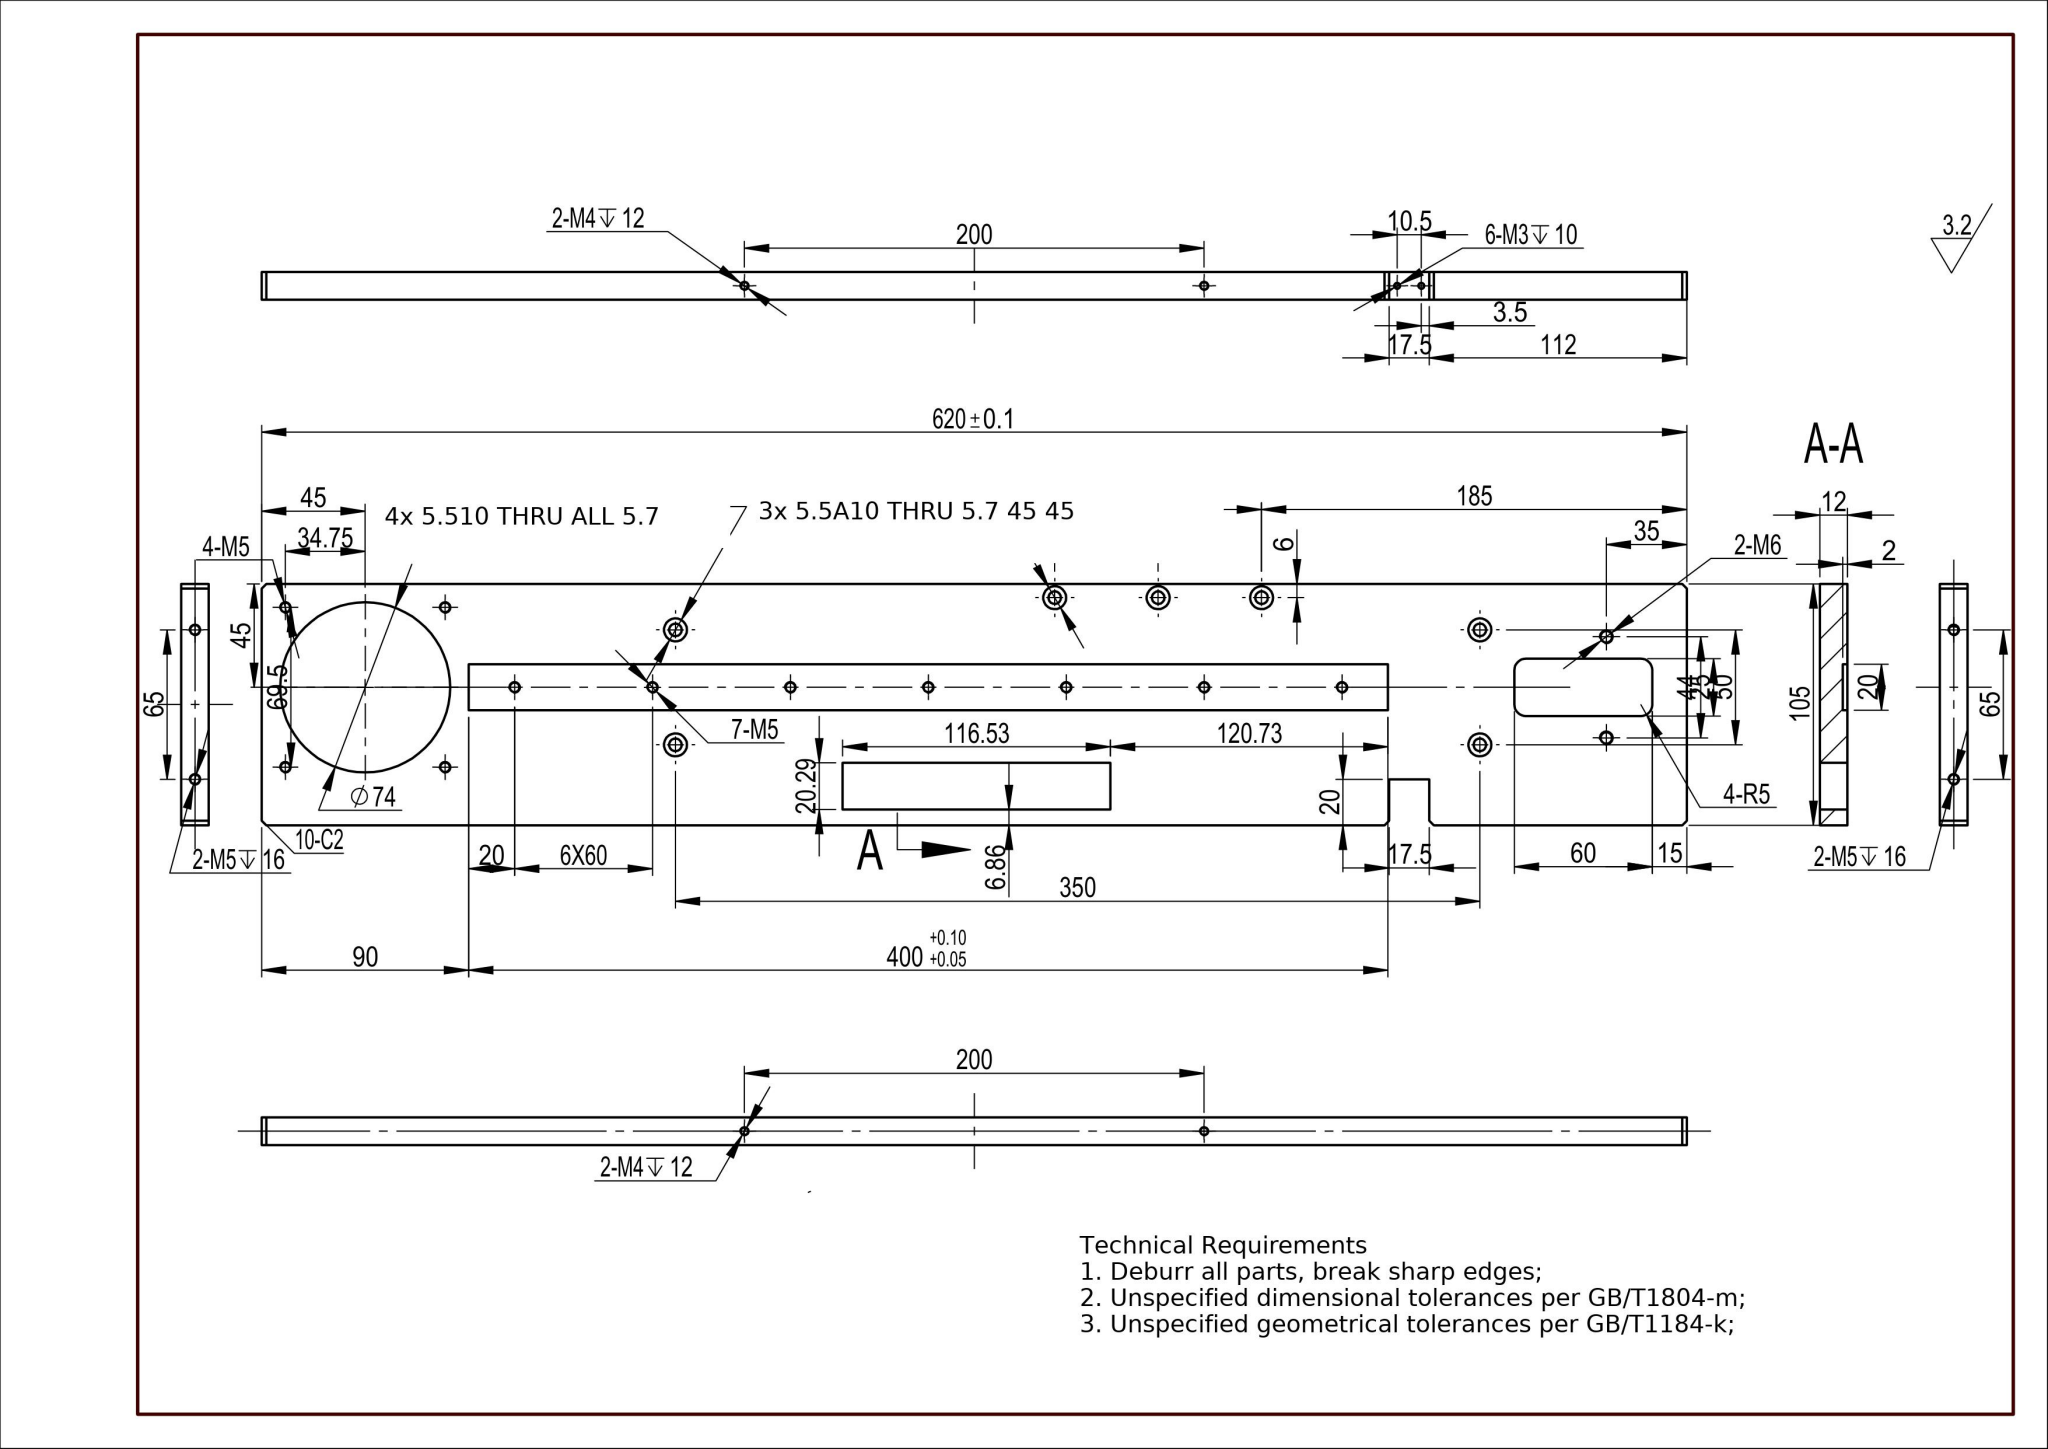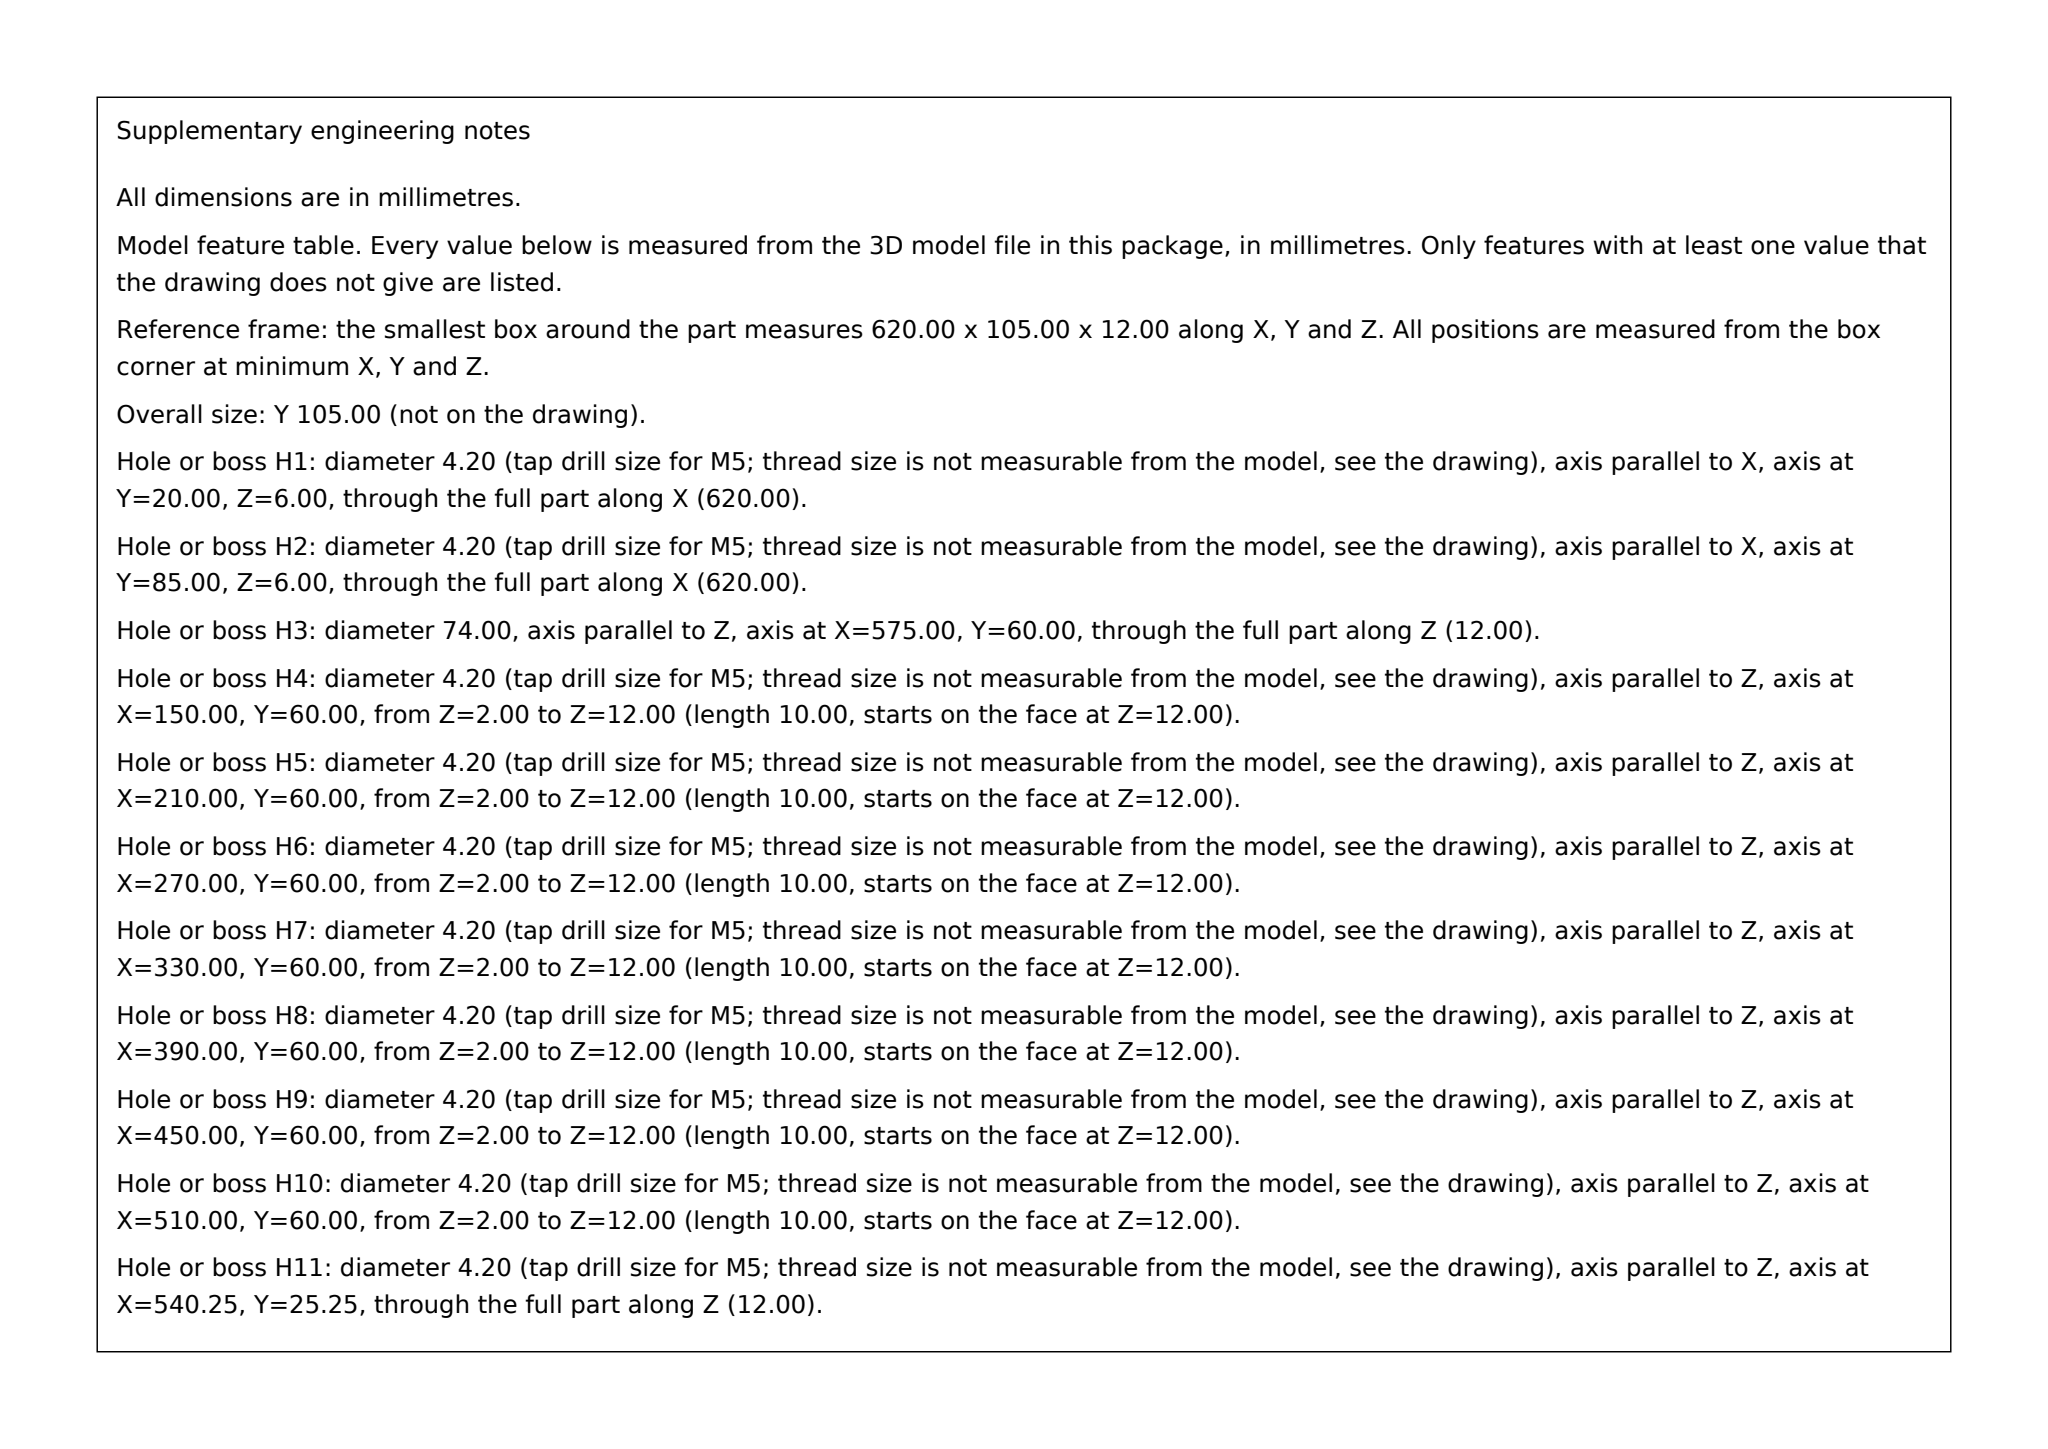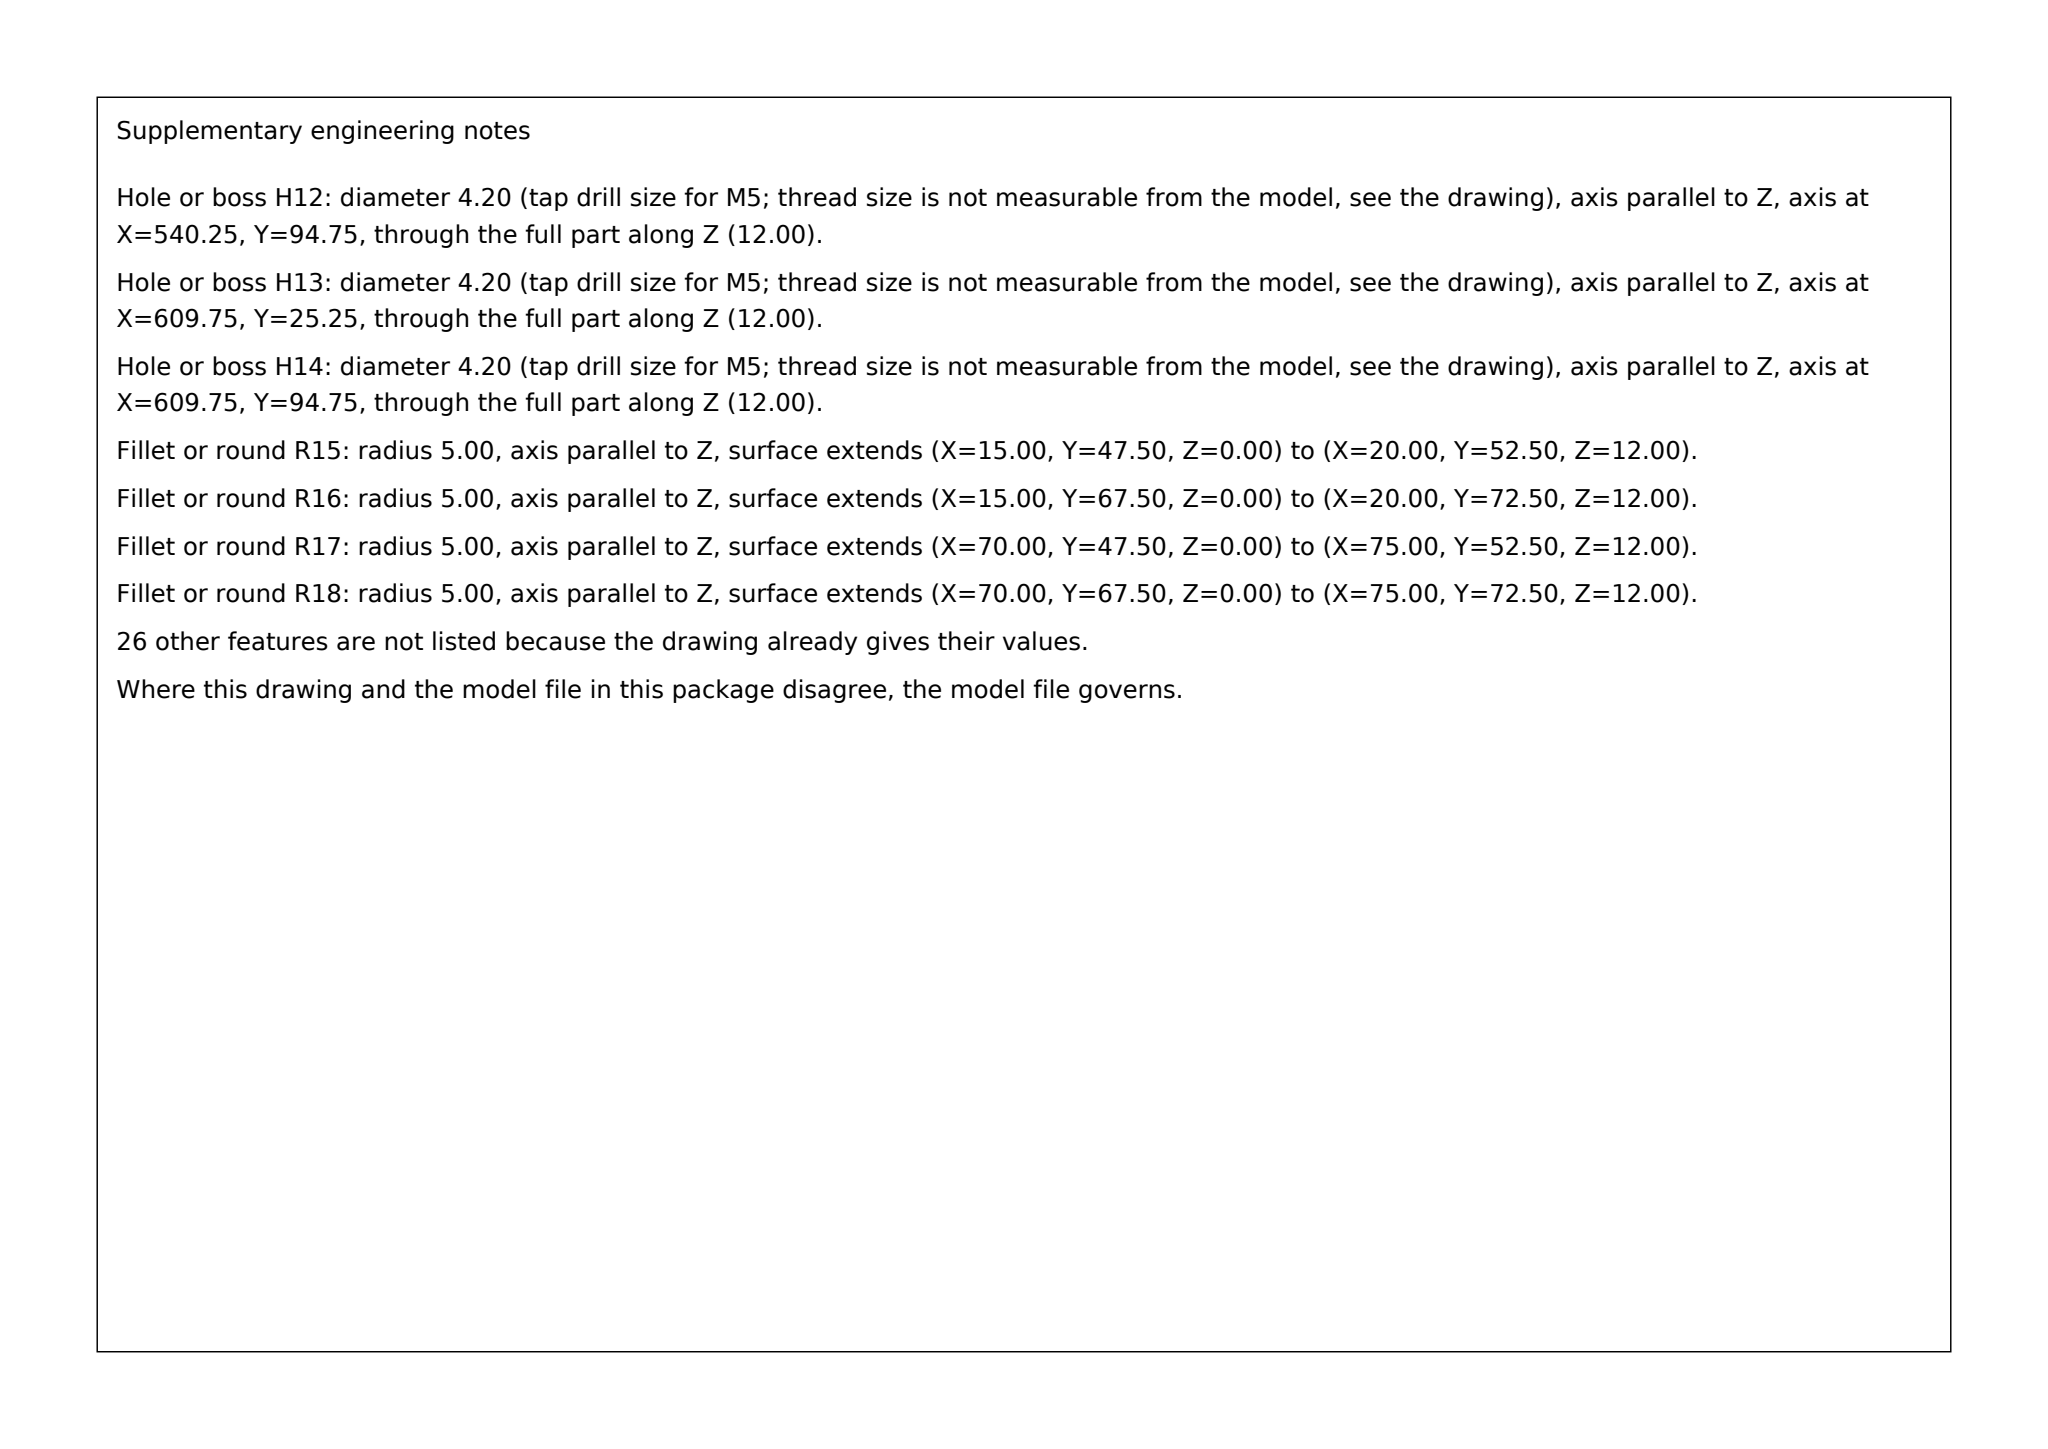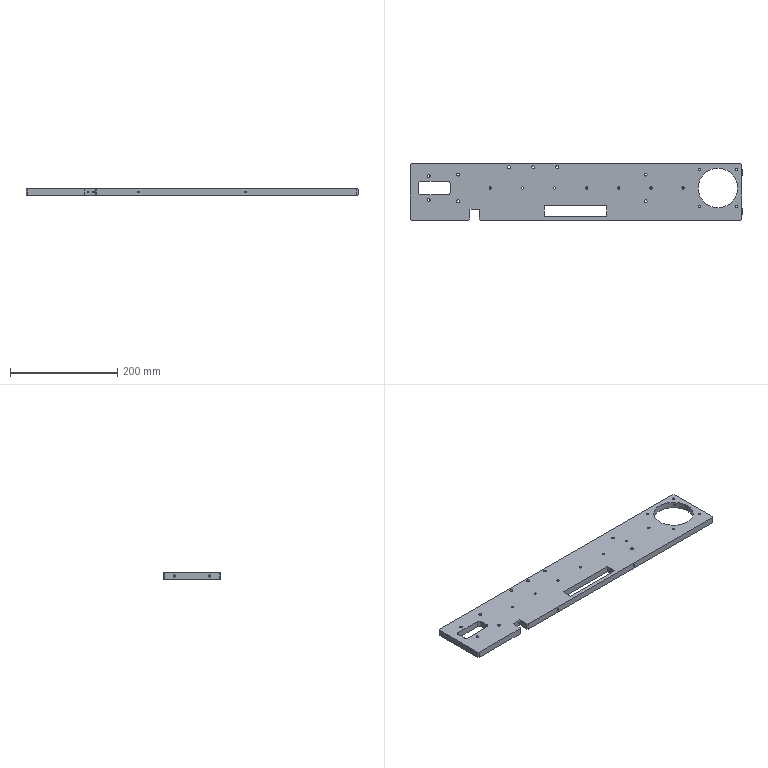Part | SolidWorks | mm | 1 solid | 135 faces | box 620 x 105 x 12 mm | volume 655163 mm3 | cylinder 80 | plane 36 | cone 19 | commonest cylinder face diameters 4.2 x30 10 x18 5.5 x14 3.3 x8 2.5 x4 5 x4 74 x2
build123d program:
from build123d import *

# Parameters (mm, degrees)
SKETCH1_W                                            = 620
SKETCH1_H                                            = 90
BOSS_EXTRUDE1_DEPTH                                  = 6
SKETCH5_R                                            = 37
CUT_EXTRUDE1_DEPTH                                   = 314.479
M5_TAPPED_HOLE1_D                                    = 4.2
M5_TAPPED_HOLE1_DEPTH                                = 17.4
M5_TAPPED_HOLE1_TIP                                  = 1.262
SKETCH6_W                                            = 400
SKETCH6_H                                            = 20
CUT_EXTRUDE2_DEPTH                                   = 2
SKETCH7_W                                            = 60
SKETCH7_H                                            = 25
CUT_EXTRUDE3_DEPTH                                   = 314.479
M6_TAPPED_HOLE1_D                                    = 5
HOLE_SIZE_ACCORDING_TO_HEX_SOCKET_HEAD_C_D           = 5.5
HOLE_SIZE_ACCORDING_TO_HEX_SOCKET_HEAD_C_CBORE_D     = 10
HOLE_SIZE_ACCORDING_TO_HEX_SOCKET_HEAD_C_CBORE_DEPTH = 5.7
HOLE_SIZE_ACCORDING_TO_HEX_SOCKET_HE_2_D             = 5.5
HOLE_SIZE_ACCORDING_TO_HEX_SOCKET_HE_2_CBORE_D       = 10
HOLE_SIZE_ACCORDING_TO_HEX_SOCKET_HE_2_CBORE_DEPTH   = 5.7
M5_TAPPED_HOLE3_D                                    = 4.2
LPATTERN1_COUNT                                      = 7
LPATTERN1_PITCH                                      = 60
SKETCH20_W                                           = 620
SKETCH20_H                                           = 12
BOSS_EXTRUDE2_DEPTH                                  = 15
M5_TAPPED_HOLE4_AT_2_COUNT                           = 2
M5_TAPPED_HOLE4_AT_2_PITCH                           = 65
SKETCH25_W                                           = 17.5
SKETCH25_H                                           = 165.922
CUT_EXTRUDE4_DEPTH                                   = 20
M4_TAPPED_HOLE1_D                                    = 3.3
M4_TAPPED_HOLE1_DEPTH                                = 15.5
M4_TAPPED_HOLE1_TIP                                  = 0.9914
M4_TAPPED_HOLE2_D                                    = 3.3
M4_TAPPED_HOLE2_DEPTH                                = 15.5
M4_TAPPED_HOLE2_TIP                                  = 0.9914
M3_TAPPED_HOLE1_D                                    = 2.5
M3_TAPPED_HOLE1_DEPTH                                = 8.5
M3_TAPPED_HOLE1_TIP                                  = 0.7511
FILLET1_R                                            = 5
CHAMFER1_SIZE                                        = 2
SKETCH32_W                                           = 116.527
SKETCH32_H                                           = 20.291
CUT_EXTRUDE5_DEPTH                                   = 80


with BuildPart() as part:
    # Sketch1 → Boss-Extrude1 (new, symmetric)
    with BuildSketch(Plane.XY):
        Rectangle(SKETCH1_W, SKETCH1_H)
    extrude(amount=BOSS_EXTRUDE1_DEPTH, both=True)

    # Sketch5 → Cut-Extrude1 (cut, through all)
    with BuildSketch(Plane.XY.offset(6)):
        with Locations((265, 0)):
            Circle(SKETCH5_R)
    extrude(amount=-CUT_EXTRUDE1_DEPTH, mode=Mode.SUBTRACT)

    # M5 Tapped Hole1
    with Locations(Plane(origin=(-53.335, 23.45, -6), x_dir=(1, 0, 0), z_dir=(0, 0, -1))):
        with Locations((353.085, -11.3), (353.085, 58.2), (283.585, 58.2), (283.585, -11.3)):
            Hole(M5_TAPPED_HOLE1_D / 2, depth=M5_TAPPED_HOLE1_DEPTH)
            with Locations((0, 0, -(M5_TAPPED_HOLE1_DEPTH + M5_TAPPED_HOLE1_TIP / 2))):  # 118° drill point
                Cone(0, M5_TAPPED_HOLE1_D / 2, M5_TAPPED_HOLE1_TIP, mode=Mode.SUBTRACT)

    # Sketch6 → Cut-Extrude2 (cut)
    with BuildSketch(Plane.XY.offset(-6)):
        with Locations((20, 0)):
            Rectangle(SKETCH6_W, SKETCH6_H)
    extrude(amount=CUT_EXTRUDE2_DEPTH, mode=Mode.SUBTRACT)

    # Sketch7 → Cut-Extrude3 (cut, through all)
    with BuildSketch(Plane.XY.offset(6)):
        with Locations((-265, 0)):
            Rectangle(SKETCH7_W, SKETCH7_H)
    extrude(amount=-CUT_EXTRUDE3_DEPTH, mode=Mode.SUBTRACT)

    # M6 Tapped Hole1 (through all)
    with Locations(Plane(origin=(-2.516, 33.465, -6), x_dir=(1, 0, 0), z_dir=(0, 0, -1))):
        with Locations((-272.484, 11.465), (-272.484, 55.465)):
            Hole(M6_TAPPED_HOLE1_D / 2)

    # Hole Size according to Hex Socket Head C (through all)
    with Locations(Plane(origin=(0, 0, -6), x_dir=(-1, 0, 0), z_dir=(0, 0, -1))):
        with Locations((220, 25), (220, -25), (-130, 25), (-130, -25)):
            CounterBoreHole(HOLE_SIZE_ACCORDING_TO_HEX_SOCKET_HEAD_C_D / 2, HOLE_SIZE_ACCORDING_TO_HEX_SOCKET_HEAD_C_CBORE_D / 2, HOLE_SIZE_ACCORDING_TO_HEX_SOCKET_HEAD_C_CBORE_DEPTH)

    # Hole Size according to Hex Socket He 2 (through all)
    with Locations(Plane(origin=(0, 0, -6), x_dir=(-1, 0, 0), z_dir=(0, 0, -1))):
        with Locations((125, 39), (80, 39), (35, 39)):
            CounterBoreHole(HOLE_SIZE_ACCORDING_TO_HEX_SOCKET_HE_2_D / 2, HOLE_SIZE_ACCORDING_TO_HEX_SOCKET_HE_2_CBORE_D / 2, HOLE_SIZE_ACCORDING_TO_HEX_SOCKET_HE_2_CBORE_DEPTH)

    # M5 Tapped Hole3 (through all)
    with Locations(Plane(origin=(0, 0, -4), x_dir=(-1, 0, 0), z_dir=(0, 0, -1))):
        with Locations((-200, 0)):
            m5_tapped_hole3 = Hole(M5_TAPPED_HOLE3_D / 2)

    # LPattern1: M5 Tapped Hole3 ×7
    with Locations(*[(-i * LPATTERN1_PITCH, 0, 0) for i in range(1, LPATTERN1_COUNT)]):
        add(m5_tapped_hole3, mode=Mode.SUBTRACT)

    # Sketch20 → Boss-Extrude2 (add)
    with BuildSketch(Plane.XZ.offset(45)):
        Rectangle(SKETCH20_W, SKETCH20_H)
    extrude(amount=BOSS_EXTRUDE2_DEPTH)

    # Sketch23 → M5 Tapped Hole4 (revolve, cut)
    with BuildSketch(Plane(origin=(-310, 25, 0), x_dir=(0, 0, 1), z_dir=(0, 1, 0))):
        Polygon((0, 0), (0, 20.262), (2.1, 19), (2.1, 0), align=None)
    m5_tapped_hole4 = revolve(axis=Axis((-316.35, 25, 0), (1, 0, 0)), mode=Mode.SUBTRACT)

    # M5 Tapped Hole4 at 2: M5 Tapped Hole4 ×2
    with Locations(*[(0, -i * M5_TAPPED_HOLE4_AT_2_PITCH, 0) for i in range(1, M5_TAPPED_HOLE4_AT_2_COUNT)]):
        add(m5_tapped_hole4, mode=Mode.SUBTRACT)

    # Mirror1: M5 Tapped Hole4 across plane
    add(m5_tapped_hole4.mirror(Plane(origin=(0, 0, 0), x_dir=(0, 0, 1), z_dir=(1, 0, 0))), mode=Mode.SUBTRACT)

    # Mirror1 copy 1 sketch → Mirror1 copy 1 (revolve, cut)
    with BuildSketch(Plane(origin=(310, -40, 0), x_dir=(0, 0, 1), z_dir=(0, 1, 0))):
        Polygon((0, 0), (0, -20.262), (2.1, -19), (2.1, 0), align=None)
    revolve(axis=Axis((316.35, -40, 0), (1, 0, 0)), mode=Mode.SUBTRACT)

    # Sketch25 → Cut-Extrude4 (cut)
    with BuildSketch(Plane.XZ.offset(60)):
        with Locations((-189.25, -5.205)):
            Rectangle(SKETCH25_W, SKETCH25_H)
    extrude(amount=-CUT_EXTRUDE4_DEPTH, mode=Mode.SUBTRACT)

    # M4 Tapped Hole1
    with Locations(Plane.XZ.offset(60)):
        with Locations((-100, 0), (100, 0)):
            Hole(M4_TAPPED_HOLE1_D / 2, depth=M4_TAPPED_HOLE1_DEPTH)
            with Locations((0, 0, -(M4_TAPPED_HOLE1_DEPTH + M4_TAPPED_HOLE1_TIP / 2))):  # 118° drill point
                Cone(0, M4_TAPPED_HOLE1_D / 2, M4_TAPPED_HOLE1_TIP, mode=Mode.SUBTRACT)

    # M4 Tapped Hole2
    with Locations(Plane(origin=(0, 45, 0), x_dir=(-1, 0, 0), z_dir=(0, 1, 0))):
        with Locations((100, 0), (-100, 0)):
            Hole(M4_TAPPED_HOLE2_D / 2, depth=M4_TAPPED_HOLE2_DEPTH)
            with Locations((0, 0, -(M4_TAPPED_HOLE2_DEPTH + M4_TAPPED_HOLE2_TIP / 2))):  # 118° drill point
                Cone(0, M4_TAPPED_HOLE2_D / 2, M4_TAPPED_HOLE2_TIP, mode=Mode.SUBTRACT)

    # M3 Tapped Hole1
    with Locations(Plane.XZ.offset(40)):
        with Locations((-194.5, 0), (-184, 0)):
            Hole(M3_TAPPED_HOLE1_D / 2, depth=M3_TAPPED_HOLE1_DEPTH)
            with Locations((0, 0, -(M3_TAPPED_HOLE1_DEPTH + M3_TAPPED_HOLE1_TIP / 2))):  # 118° drill point
                Cone(0, M3_TAPPED_HOLE1_D / 2, M3_TAPPED_HOLE1_TIP, mode=Mode.SUBTRACT)

    # Fillet1
    fillet1_edges = [part.edges().sort_by_distance(p)[0] for p in [
        (-295, -12.5, 0),
        (-295, 12.5, 0),
        (-235, 12.5, 0),
        (-235, -12.5, 0),
    ]]
    fillet(fillet1_edges, radius=FILLET1_R)

    # Chamfer1
    chamfer1_edges = [part.edges().sort_by_distance(p)[0] for p in [
        (-310, -60, 0),
        (310, -60, 0),
        (-180.5, -60, 0),
        (-198, -60, 0),
        (-310, 45, 0),
        (310, 45, 0),
    ]]
    chamfer(chamfer1_edges, length=CHAMFER1_SIZE)

    # Sketch32 → Cut-Extrude5 (cut)
    with BuildSketch(Plane.XY.offset(6)):
        with Locations((-1.003, -42.994)):
            Rectangle(SKETCH32_W, SKETCH32_H)
    extrude(amount=-CUT_EXTRUDE5_DEPTH, mode=Mode.SUBTRACT)


solid = part.part